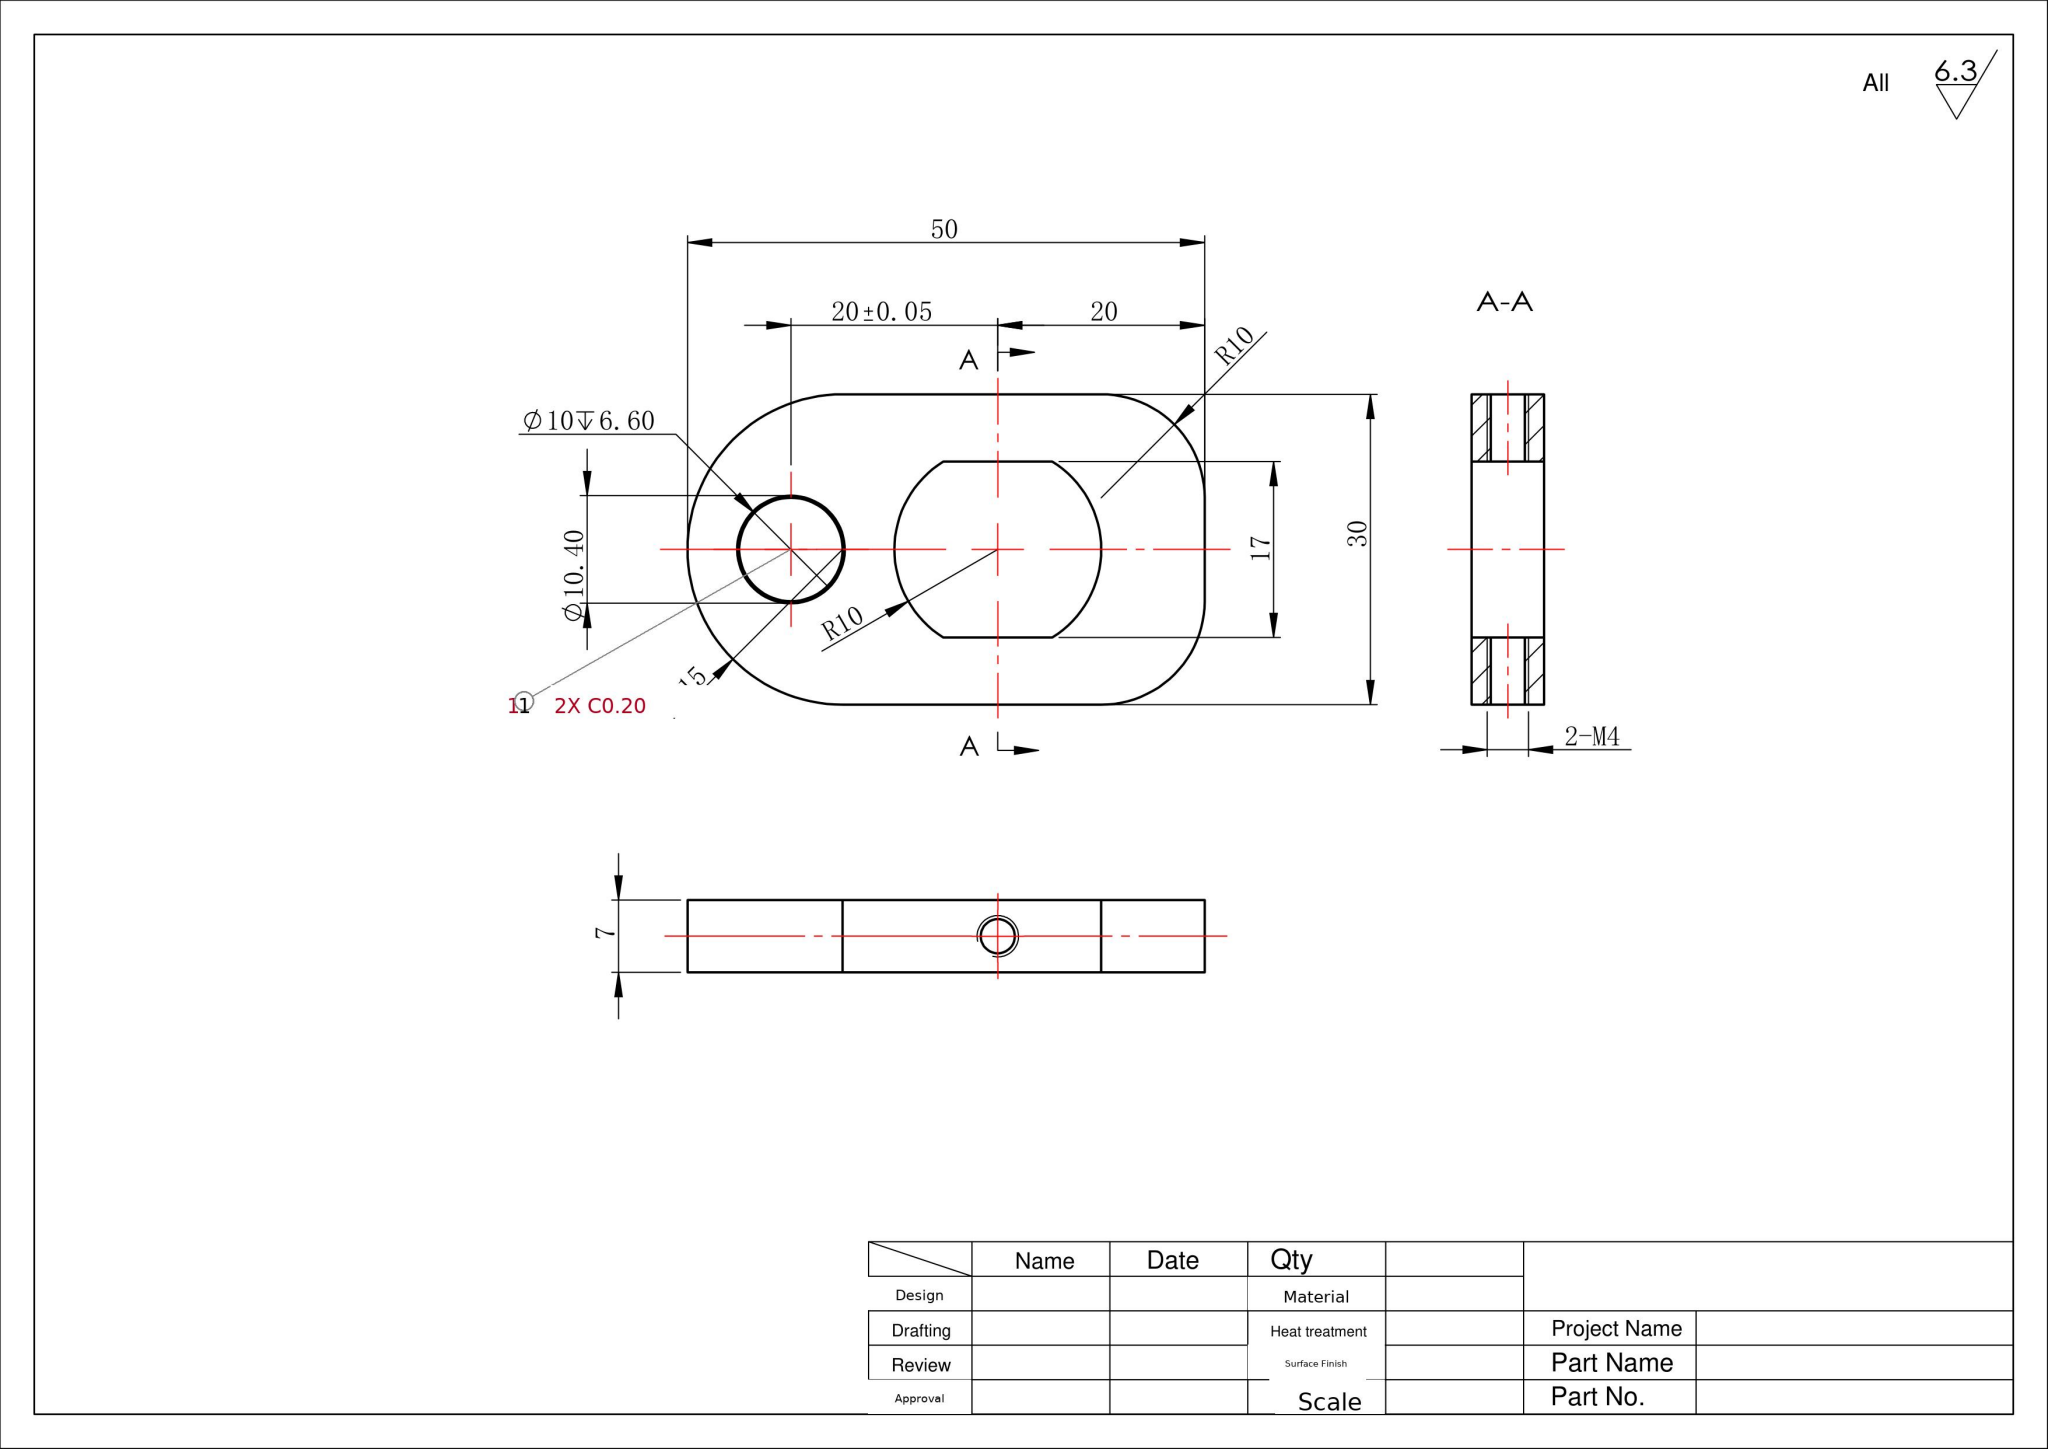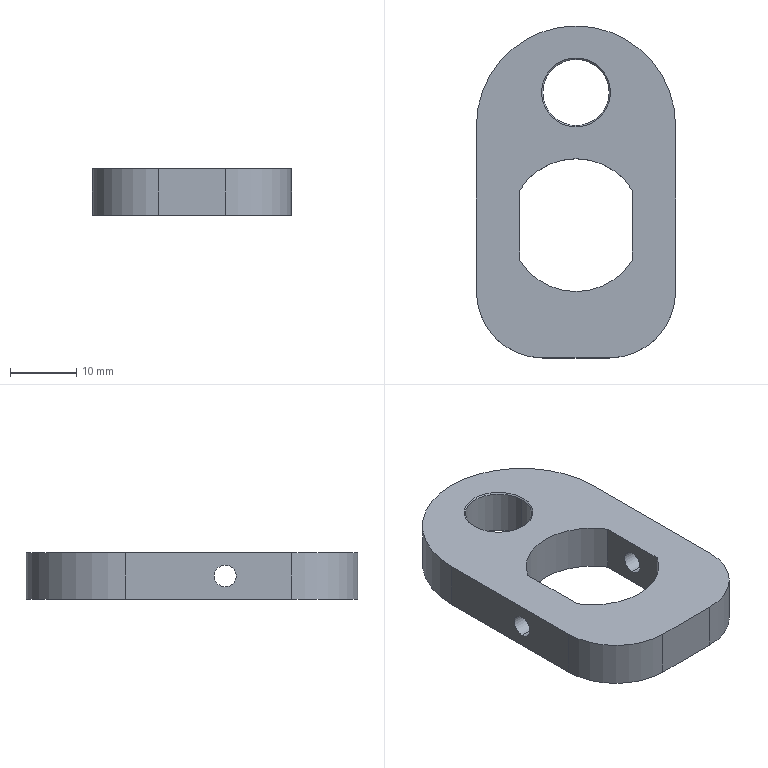Part | SolidWorks | mm | 1 solid | 23 faces | box 30 x 50 x 7 mm | volume 6812 mm3 | cylinder 12 | plane 7 | cone 4 | commonest cylinder face diameters 3.3 x4 20 x4 10 x2 30 x2
STEP:
#1=CARTESIAN_POINT('',(5.,20.,0.2));
#2=VERTEX_POINT('',#1);
#3=CARTESIAN_POINT('',(-5.,20.,0.2));
#4=VERTEX_POINT('',#3);
#5=CARTESIAN_POINT('',(-0.,20.,0.2));
#6=DIRECTION('',(0.,0.,-1.));
#7=DIRECTION('',(-1.,0.,0.));
#8=AXIS2_PLACEMENT_3D('',#5,#6,#7);
#9=CIRCLE('',#8,5.);
#10=EDGE_CURVE('',#2,#4,#9,.T.);
#11=ORIENTED_EDGE('',*,*,#10,.F.);
#12=CARTESIAN_POINT('',(5.2,20.,0.));
#13=VERTEX_POINT('',#12);
#14=CARTESIAN_POINT('',(5.,20.,0.2));
#15=DIRECTION('',(0.7071,0.,-0.7071));
#16=VECTOR('',#15,1000.);
#17=LINE('',#14,#16);
#18=EDGE_CURVE('',#2,#13,#17,.T.);
#19=ORIENTED_EDGE('',*,*,#18,.T.);
#20=CARTESIAN_POINT('',(-5.2,20.,0.));
#21=VERTEX_POINT('',#20);
#22=CARTESIAN_POINT('',(-0.,20.,0.));
#23=DIRECTION('',(0.,0.,1.));
#24=DIRECTION('',(-1.,0.,0.));
#25=AXIS2_PLACEMENT_3D('',#22,#23,#24);
#26=CIRCLE('',#25,5.2);
#27=EDGE_CURVE('',#21,#13,#26,.T.);
#28=ORIENTED_EDGE('',*,*,#27,.F.);
#29=CARTESIAN_POINT('',(-5.,20.,0.2));
#30=DIRECTION('',(-0.7071,0.,-0.7071));
#31=VECTOR('',#30,1000.);
#32=LINE('',#29,#31);
#33=EDGE_CURVE('',#4,#21,#32,.T.);
#34=ORIENTED_EDGE('',*,*,#33,.F.);
#35=EDGE_LOOP('',(#11,#19,#28,#34));
#36=FACE_OUTER_BOUND('',#35,.T.);
#37=CARTESIAN_POINT('',(-0.,20.,0.2));
#38=DIRECTION('',(0.,0.,-1.));
#39=DIRECTION('',(-1.,0.,0.));
#40=AXIS2_PLACEMENT_3D('',#37,#38,#39);
#41=CONICAL_SURFACE('',#40,5.,0.7854);
#42=ADVANCED_FACE('',(#36),#41,.F.);
#43=CARTESIAN_POINT('',(-5.,20.,6.8));
#44=VERTEX_POINT('',#43);
#45=CARTESIAN_POINT('',(5.,20.,6.8));
#46=VERTEX_POINT('',#45);
#47=CARTESIAN_POINT('',(-0.,20.,6.8));
#48=DIRECTION('',(0.,0.,1.));
#49=DIRECTION('',(-1.,0.,0.));
#50=AXIS2_PLACEMENT_3D('',#47,#48,#49);
#51=CIRCLE('',#50,5.);
#52=EDGE_CURVE('',#44,#46,#51,.T.);
#53=ORIENTED_EDGE('',*,*,#52,.F.);
#54=CARTESIAN_POINT('',(-5.2,20.,7.));
#55=VERTEX_POINT('',#54);
#56=CARTESIAN_POINT('',(-5.2,20.,7.));
#57=DIRECTION('',(-0.7071,0.,0.7071));
#58=VECTOR('',#57,1000.);
#59=LINE('',#56,#58);
#60=EDGE_CURVE('',#44,#55,#59,.T.);
#61=ORIENTED_EDGE('',*,*,#60,.T.);
#62=CARTESIAN_POINT('',(5.2,20.,7.));
#63=VERTEX_POINT('',#62);
#64=CARTESIAN_POINT('',(-0.,20.,7.));
#65=DIRECTION('',(0.,0.,-1.));
#66=DIRECTION('',(-1.,0.,0.));
#67=AXIS2_PLACEMENT_3D('',#64,#65,#66);
#68=CIRCLE('',#67,5.2);
#69=EDGE_CURVE('',#63,#55,#68,.T.);
#70=ORIENTED_EDGE('',*,*,#69,.F.);
#71=CARTESIAN_POINT('',(5.2,20.,7.));
#72=DIRECTION('',(0.7071,0.,0.7071));
#73=VECTOR('',#72,1000.);
#74=LINE('',#71,#73);
#75=EDGE_CURVE('',#46,#63,#74,.T.);
#76=ORIENTED_EDGE('',*,*,#75,.F.);
#77=EDGE_LOOP('',(#53,#61,#70,#76));
#78=FACE_OUTER_BOUND('',#77,.T.);
#79=CARTESIAN_POINT('',(-0.,20.,7.));
#80=DIRECTION('',(0.,0.,1.));
#81=DIRECTION('',(1.,0.,0.));
#82=AXIS2_PLACEMENT_3D('',#79,#80,#81);
#83=CONICAL_SURFACE('',#82,5.2,0.7854);
#84=ADVANCED_FACE('',(#78),#83,.F.);
#85=CARTESIAN_POINT('',(15.,0.,1.85));
#86=VERTEX_POINT('',#85);
#87=CARTESIAN_POINT('',(15.,0.,5.15));
#88=VERTEX_POINT('',#87);
#89=CARTESIAN_POINT('',(15.,0.,3.5));
#90=DIRECTION('',(-1.,0.,0.));
#91=DIRECTION('',(0.,0.,1.));
#92=AXIS2_PLACEMENT_3D('',#89,#90,#91);
#93=CIRCLE('',#92,1.65);
#94=EDGE_CURVE('',#86,#88,#93,.T.);
#95=ORIENTED_EDGE('',*,*,#94,.F.);
#96=CARTESIAN_POINT('',(8.5,0.,1.85));
#97=VERTEX_POINT('',#96);
#98=CARTESIAN_POINT('',(-15.,0.,1.85));
#99=DIRECTION('',(-1.,0.,0.));
#100=VECTOR('',#99,1000.);
#101=LINE('',#98,#100);
#102=EDGE_CURVE('',#86,#97,#101,.T.);
#103=ORIENTED_EDGE('',*,*,#102,.T.);
#104=CARTESIAN_POINT('',(8.5,0.,5.15));
#105=VERTEX_POINT('',#104);
#106=CARTESIAN_POINT('',(8.5,0.,3.5));
#107=DIRECTION('',(-1.,0.,0.));
#108=DIRECTION('',(0.,-1.,0.));
#109=AXIS2_PLACEMENT_3D('',#106,#107,#108);
#110=CIRCLE('',#109,1.65);
#111=EDGE_CURVE('',#97,#105,#110,.T.);
#112=ORIENTED_EDGE('',*,*,#111,.T.);
#113=CARTESIAN_POINT('',(-15.,0.,5.15));
#114=DIRECTION('',(-1.,0.,0.));
#115=VECTOR('',#114,1000.);
#116=LINE('',#113,#115);
#117=EDGE_CURVE('',#88,#105,#116,.T.);
#118=ORIENTED_EDGE('',*,*,#117,.F.);
#119=EDGE_LOOP('',(#95,#103,#112,#118));
#120=FACE_OUTER_BOUND('',#119,.T.);
#121=CARTESIAN_POINT('',(-15.,0.,3.5));
#122=DIRECTION('',(-1.,0.,0.));
#123=DIRECTION('',(0.,0.,1.));
#124=AXIS2_PLACEMENT_3D('',#121,#122,#123);
#125=CYLINDRICAL_SURFACE('',#124,1.65);
#126=ADVANCED_FACE('',(#120),#125,.F.);
#127=CARTESIAN_POINT('',(-8.5,0.,5.15));
#128=VERTEX_POINT('',#127);
#129=CARTESIAN_POINT('',(-8.5,0.,1.85));
#130=VERTEX_POINT('',#129);
#131=CARTESIAN_POINT('',(-8.5,0.,3.5));
#132=DIRECTION('',(1.,0.,0.));
#133=DIRECTION('',(0.,1.,0.));
#134=AXIS2_PLACEMENT_3D('',#131,#132,#133);
#135=CIRCLE('',#134,1.65);
#136=EDGE_CURVE('',#128,#130,#135,.T.);
#137=ORIENTED_EDGE('',*,*,#136,.T.);
#138=CARTESIAN_POINT('',(-15.,0.,1.85));
#139=VERTEX_POINT('',#138);
#140=CARTESIAN_POINT('',(-15.,0.,1.85));
#141=DIRECTION('',(-1.,0.,0.));
#142=VECTOR('',#141,1000.);
#143=LINE('',#140,#142);
#144=EDGE_CURVE('',#130,#139,#143,.T.);
#145=ORIENTED_EDGE('',*,*,#144,.T.);
#146=CARTESIAN_POINT('',(-15.,0.,5.15));
#147=VERTEX_POINT('',#146);
#148=CARTESIAN_POINT('',(-15.,0.,3.5));
#149=DIRECTION('',(-1.,0.,0.));
#150=DIRECTION('',(0.,0.,1.));
#151=AXIS2_PLACEMENT_3D('',#148,#149,#150);
#152=CIRCLE('',#151,1.65);
#153=EDGE_CURVE('',#139,#147,#152,.T.);
#154=ORIENTED_EDGE('',*,*,#153,.T.);
#155=CARTESIAN_POINT('',(-15.,0.,5.15));
#156=DIRECTION('',(-1.,0.,0.));
#157=VECTOR('',#156,1000.);
#158=LINE('',#155,#157);
#159=EDGE_CURVE('',#128,#147,#158,.T.);
#160=ORIENTED_EDGE('',*,*,#159,.F.);
#161=EDGE_LOOP('',(#137,#145,#154,#160));
#162=FACE_OUTER_BOUND('',#161,.T.);
#163=CARTESIAN_POINT('',(-15.,0.,3.5));
#164=DIRECTION('',(-1.,0.,0.));
#165=DIRECTION('',(0.,0.,1.));
#166=AXIS2_PLACEMENT_3D('',#163,#164,#165);
#167=CYLINDRICAL_SURFACE('',#166,1.65);
#168=ADVANCED_FACE('',(#162),#167,.F.);
#169=ORIENTED_EDGE('',*,*,#52,.T.);
#170=CARTESIAN_POINT('',(5.,20.,7.));
#171=DIRECTION('',(0.,0.,-1.));
#172=VECTOR('',#171,1000.);
#173=LINE('',#170,#172);
#174=EDGE_CURVE('',#46,#2,#173,.T.);
#175=ORIENTED_EDGE('',*,*,#174,.T.);
#176=ORIENTED_EDGE('',*,*,#10,.T.);
#177=CARTESIAN_POINT('',(-5.,20.,7.));
#178=DIRECTION('',(0.,0.,-1.));
#179=VECTOR('',#178,1000.);
#180=LINE('',#177,#179);
#181=EDGE_CURVE('',#44,#4,#180,.T.);
#182=ORIENTED_EDGE('',*,*,#181,.F.);
#183=EDGE_LOOP('',(#169,#175,#176,#182));
#184=FACE_OUTER_BOUND('',#183,.T.);
#185=CARTESIAN_POINT('',(-0.,20.,7.));
#186=DIRECTION('',(0.,0.,-1.));
#187=DIRECTION('',(-1.,0.,0.));
#188=AXIS2_PLACEMENT_3D('',#185,#186,#187);
#189=CYLINDRICAL_SURFACE('',#188,5.);
#190=ADVANCED_FACE('',(#184),#189,.F.);
#191=ORIENTED_EDGE('',*,*,#69,.T.);
#192=CARTESIAN_POINT('',(-0.,20.,7.));
#193=DIRECTION('',(0.,0.,-1.));
#194=DIRECTION('',(-1.,0.,0.));
#195=AXIS2_PLACEMENT_3D('',#192,#193,#194);
#196=CIRCLE('',#195,5.2);
#197=EDGE_CURVE('',#55,#63,#196,.T.);
#198=ORIENTED_EDGE('',*,*,#197,.T.);
#199=EDGE_LOOP('',(#191,#198));
#200=FACE_BOUND('',#199,.T.);
#201=CARTESIAN_POINT('',(-15.,15.,7.));
#202=VERTEX_POINT('',#201);
#203=CARTESIAN_POINT('',(-15.,-10.,7.));
#204=VERTEX_POINT('',#203);
#205=CARTESIAN_POINT('',(-15.,-30.,7.));
#206=DIRECTION('',(0.,-1.,0.));
#207=VECTOR('',#206,1000.);
#208=LINE('',#205,#207);
#209=EDGE_CURVE('',#202,#204,#208,.T.);
#210=ORIENTED_EDGE('',*,*,#209,.T.);
#211=CARTESIAN_POINT('',(-5.,-20.,7.));
#212=VERTEX_POINT('',#211);
#213=CARTESIAN_POINT('',(-5.,-10.,7.));
#214=DIRECTION('',(0.,0.,1.));
#215=DIRECTION('',(-1.,0.,0.));
#216=AXIS2_PLACEMENT_3D('',#213,#214,#215);
#217=CIRCLE('',#216,10.);
#218=EDGE_CURVE('',#204,#212,#217,.T.);
#219=ORIENTED_EDGE('',*,*,#218,.T.);
#220=CARTESIAN_POINT('',(5.,-20.,7.));
#221=VERTEX_POINT('',#220);
#222=CARTESIAN_POINT('',(29.445,-20.,7.));
#223=DIRECTION('',(1.,0.,0.));
#224=VECTOR('',#223,1000.);
#225=LINE('',#222,#224);
#226=EDGE_CURVE('',#212,#221,#225,.T.);
#227=ORIENTED_EDGE('',*,*,#226,.T.);
#228=CARTESIAN_POINT('',(15.,-10.,7.));
#229=VERTEX_POINT('',#228);
#230=CARTESIAN_POINT('',(5.,-10.,7.));
#231=DIRECTION('',(0.,0.,1.));
#232=DIRECTION('',(-1.,0.,0.));
#233=AXIS2_PLACEMENT_3D('',#230,#231,#232);
#234=CIRCLE('',#233,10.);
#235=EDGE_CURVE('',#221,#229,#234,.T.);
#236=ORIENTED_EDGE('',*,*,#235,.T.);
#237=CARTESIAN_POINT('',(15.,15.,7.));
#238=VERTEX_POINT('',#237);
#239=CARTESIAN_POINT('',(15.,-30.,7.));
#240=DIRECTION('',(0.,1.,0.));
#241=VECTOR('',#240,1000.);
#242=LINE('',#239,#241);
#243=EDGE_CURVE('',#229,#238,#242,.T.);
#244=ORIENTED_EDGE('',*,*,#243,.T.);
#245=CARTESIAN_POINT('',(0.,30.,7.));
#246=VERTEX_POINT('',#245);
#247=CARTESIAN_POINT('',(0.,15.,7.));
#248=DIRECTION('',(0.,0.,1.));
#249=DIRECTION('',(-1.,0.,0.));
#250=AXIS2_PLACEMENT_3D('',#247,#248,#249);
#251=CIRCLE('',#250,15.);
#252=EDGE_CURVE('',#238,#246,#251,.T.);
#253=ORIENTED_EDGE('',*,*,#252,.T.);
#254=CARTESIAN_POINT('',(0.,15.,7.));
#255=DIRECTION('',(0.,0.,1.));
#256=DIRECTION('',(-1.,0.,0.));
#257=AXIS2_PLACEMENT_3D('',#254,#255,#256);
#258=CIRCLE('',#257,15.);
#259=EDGE_CURVE('',#246,#202,#258,.T.);
#260=ORIENTED_EDGE('',*,*,#259,.T.);
#261=EDGE_LOOP('',(#210,#219,#227,#236,#244,#253,#260));
#262=FACE_OUTER_BOUND('',#261,.T.);
#263=CARTESIAN_POINT('',(-8.5,-5.268,7.));
#264=VERTEX_POINT('',#263);
#265=CARTESIAN_POINT('',(8.5,-5.268,7.));
#266=VERTEX_POINT('',#265);
#267=CARTESIAN_POINT('',(0.,0.,7.));
#268=DIRECTION('',(0.,0.,1.));
#269=DIRECTION('',(1.,0.,0.));
#270=AXIS2_PLACEMENT_3D('',#267,#268,#269);
#271=CIRCLE('',#270,10.);
#272=EDGE_CURVE('',#264,#266,#271,.T.);
#273=ORIENTED_EDGE('',*,*,#272,.F.);
#274=CARTESIAN_POINT('',(-8.5,5.268,7.));
#275=VERTEX_POINT('',#274);
#276=CARTESIAN_POINT('',(-8.5,-5.268,7.));
#277=DIRECTION('',(0.,-1.,0.));
#278=VECTOR('',#277,1000.);
#279=LINE('',#276,#278);
#280=EDGE_CURVE('',#275,#264,#279,.T.);
#281=ORIENTED_EDGE('',*,*,#280,.F.);
#282=CARTESIAN_POINT('',(8.5,5.268,7.));
#283=VERTEX_POINT('',#282);
#284=CARTESIAN_POINT('',(0.,0.,7.));
#285=DIRECTION('',(0.,0.,1.));
#286=DIRECTION('',(1.,0.,0.));
#287=AXIS2_PLACEMENT_3D('',#284,#285,#286);
#288=CIRCLE('',#287,10.);
#289=EDGE_CURVE('',#283,#275,#288,.T.);
#290=ORIENTED_EDGE('',*,*,#289,.F.);
#291=CARTESIAN_POINT('',(8.5,-5.268,7.));
#292=DIRECTION('',(0.,1.,0.));
#293=VECTOR('',#292,1000.);
#294=LINE('',#291,#293);
#295=EDGE_CURVE('',#266,#283,#294,.T.);
#296=ORIENTED_EDGE('',*,*,#295,.F.);
#297=EDGE_LOOP('',(#273,#281,#290,#296));
#298=FACE_BOUND('',#297,.T.);
#299=CARTESIAN_POINT('',(-15.,30.,7.));
#300=DIRECTION('',(0.,0.,-1.));
#301=DIRECTION('',(-1.,0.,0.));
#302=AXIS2_PLACEMENT_3D('',#299,#300,#301);
#303=PLANE('',#302);
#304=ADVANCED_FACE('',(#200,#262,#298),#303,.F.);
#305=ORIENTED_EDGE('',*,*,#27,.T.);
#306=CARTESIAN_POINT('',(-0.,20.,0.));
#307=DIRECTION('',(0.,0.,1.));
#308=DIRECTION('',(-1.,0.,0.));
#309=AXIS2_PLACEMENT_3D('',#306,#307,#308);
#310=CIRCLE('',#309,5.2);
#311=EDGE_CURVE('',#13,#21,#310,.T.);
#312=ORIENTED_EDGE('',*,*,#311,.T.);
#313=EDGE_LOOP('',(#305,#312));
#314=FACE_BOUND('',#313,.T.);
#315=CARTESIAN_POINT('',(-5.,-20.,0.));
#316=VERTEX_POINT('',#315);
#317=CARTESIAN_POINT('',(5.,-20.,0.));
#318=VERTEX_POINT('',#317);
#319=CARTESIAN_POINT('',(29.445,-20.,0.));
#320=DIRECTION('',(1.,0.,0.));
#321=VECTOR('',#320,1000.);
#322=LINE('',#319,#321);
#323=EDGE_CURVE('',#316,#318,#322,.T.);
#324=ORIENTED_EDGE('',*,*,#323,.F.);
#325=CARTESIAN_POINT('',(-15.,-10.,0.));
#326=VERTEX_POINT('',#325);
#327=CARTESIAN_POINT('',(-5.,-10.,0.));
#328=DIRECTION('',(0.,0.,-1.));
#329=DIRECTION('',(-1.,0.,0.));
#330=AXIS2_PLACEMENT_3D('',#327,#328,#329);
#331=CIRCLE('',#330,10.);
#332=EDGE_CURVE('',#316,#326,#331,.T.);
#333=ORIENTED_EDGE('',*,*,#332,.T.);
#334=CARTESIAN_POINT('',(-15.,15.,0.));
#335=VERTEX_POINT('',#334);
#336=CARTESIAN_POINT('',(-15.,-30.,0.));
#337=DIRECTION('',(0.,-1.,0.));
#338=VECTOR('',#337,1000.);
#339=LINE('',#336,#338);
#340=EDGE_CURVE('',#335,#326,#339,.T.);
#341=ORIENTED_EDGE('',*,*,#340,.F.);
#342=CARTESIAN_POINT('',(0.,30.,0.));
#343=VERTEX_POINT('',#342);
#344=CARTESIAN_POINT('',(0.,15.,0.));
#345=DIRECTION('',(0.,0.,-1.));
#346=DIRECTION('',(-1.,0.,0.));
#347=AXIS2_PLACEMENT_3D('',#344,#345,#346);
#348=CIRCLE('',#347,15.);
#349=EDGE_CURVE('',#335,#343,#348,.T.);
#350=ORIENTED_EDGE('',*,*,#349,.T.);
#351=CARTESIAN_POINT('',(15.,15.,0.));
#352=VERTEX_POINT('',#351);
#353=CARTESIAN_POINT('',(0.,15.,0.));
#354=DIRECTION('',(0.,0.,-1.));
#355=DIRECTION('',(-1.,0.,0.));
#356=AXIS2_PLACEMENT_3D('',#353,#354,#355);
#357=CIRCLE('',#356,15.);
#358=EDGE_CURVE('',#343,#352,#357,.T.);
#359=ORIENTED_EDGE('',*,*,#358,.T.);
#360=CARTESIAN_POINT('',(15.,-10.,0.));
#361=VERTEX_POINT('',#360);
#362=CARTESIAN_POINT('',(15.,-30.,0.));
#363=DIRECTION('',(0.,1.,0.));
#364=VECTOR('',#363,1000.);
#365=LINE('',#362,#364);
#366=EDGE_CURVE('',#361,#352,#365,.T.);
#367=ORIENTED_EDGE('',*,*,#366,.F.);
#368=CARTESIAN_POINT('',(5.,-10.,0.));
#369=DIRECTION('',(0.,0.,-1.));
#370=DIRECTION('',(-1.,0.,0.));
#371=AXIS2_PLACEMENT_3D('',#368,#369,#370);
#372=CIRCLE('',#371,10.);
#373=EDGE_CURVE('',#361,#318,#372,.T.);
#374=ORIENTED_EDGE('',*,*,#373,.T.);
#375=EDGE_LOOP('',(#324,#333,#341,#350,#359,#367,#374));
#376=FACE_OUTER_BOUND('',#375,.T.);
#377=CARTESIAN_POINT('',(-8.5,5.268,0.));
#378=VERTEX_POINT('',#377);
#379=CARTESIAN_POINT('',(-8.5,-5.268,0.));
#380=VERTEX_POINT('',#379);
#381=CARTESIAN_POINT('',(-8.5,-5.268,0.));
#382=DIRECTION('',(0.,-1.,0.));
#383=VECTOR('',#382,1000.);
#384=LINE('',#381,#383);
#385=EDGE_CURVE('',#378,#380,#384,.T.);
#386=ORIENTED_EDGE('',*,*,#385,.T.);
#387=CARTESIAN_POINT('',(8.5,-5.268,0.));
#388=VERTEX_POINT('',#387);
#389=CARTESIAN_POINT('',(0.,0.,0.));
#390=DIRECTION('',(0.,0.,1.));
#391=DIRECTION('',(1.,0.,0.));
#392=AXIS2_PLACEMENT_3D('',#389,#390,#391);
#393=CIRCLE('',#392,10.);
#394=EDGE_CURVE('',#380,#388,#393,.T.);
#395=ORIENTED_EDGE('',*,*,#394,.T.);
#396=CARTESIAN_POINT('',(8.5,5.268,0.));
#397=VERTEX_POINT('',#396);
#398=CARTESIAN_POINT('',(8.5,-5.268,0.));
#399=DIRECTION('',(0.,1.,0.));
#400=VECTOR('',#399,1000.);
#401=LINE('',#398,#400);
#402=EDGE_CURVE('',#388,#397,#401,.T.);
#403=ORIENTED_EDGE('',*,*,#402,.T.);
#404=CARTESIAN_POINT('',(0.,0.,0.));
#405=DIRECTION('',(0.,0.,1.));
#406=DIRECTION('',(1.,0.,0.));
#407=AXIS2_PLACEMENT_3D('',#404,#405,#406);
#408=CIRCLE('',#407,10.);
#409=EDGE_CURVE('',#397,#378,#408,.T.);
#410=ORIENTED_EDGE('',*,*,#409,.T.);
#411=EDGE_LOOP('',(#386,#395,#403,#410));
#412=FACE_BOUND('',#411,.T.);
#413=CARTESIAN_POINT('',(-15.,30.,0.));
#414=DIRECTION('',(0.,0.,-1.));
#415=DIRECTION('',(-1.,0.,0.));
#416=AXIS2_PLACEMENT_3D('',#413,#414,#415);
#417=PLANE('',#416);
#418=ADVANCED_FACE('',(#314,#376,#412),#417,.T.);
#419=CARTESIAN_POINT('',(-15.,0.,3.5));
#420=DIRECTION('',(-1.,0.,0.));
#421=DIRECTION('',(0.,0.,1.));
#422=AXIS2_PLACEMENT_3D('',#419,#420,#421);
#423=CIRCLE('',#422,1.65);
#424=EDGE_CURVE('',#147,#139,#423,.T.);
#425=ORIENTED_EDGE('',*,*,#424,.F.);
#426=ORIENTED_EDGE('',*,*,#153,.F.);
#427=EDGE_LOOP('',(#425,#426));
#428=FACE_BOUND('',#427,.T.);
#429=ORIENTED_EDGE('',*,*,#340,.T.);
#430=CARTESIAN_POINT('',(-15.,-10.,7.));
#431=DIRECTION('',(0.,0.,1.));
#432=VECTOR('',#431,1000.);
#433=LINE('',#430,#432);
#434=EDGE_CURVE('',#326,#204,#433,.T.);
#435=ORIENTED_EDGE('',*,*,#434,.T.);
#436=ORIENTED_EDGE('',*,*,#209,.F.);
#437=CARTESIAN_POINT('',(-15.,15.,7.));
#438=DIRECTION('',(0.,0.,-1.));
#439=VECTOR('',#438,1000.);
#440=LINE('',#437,#439);
#441=EDGE_CURVE('',#202,#335,#440,.T.);
#442=ORIENTED_EDGE('',*,*,#441,.T.);
#443=EDGE_LOOP('',(#429,#435,#436,#442));
#444=FACE_OUTER_BOUND('',#443,.T.);
#445=CARTESIAN_POINT('',(-15.,-30.,7.));
#446=DIRECTION('',(1.,0.,0.));
#447=DIRECTION('',(0.,0.,-1.));
#448=AXIS2_PLACEMENT_3D('',#445,#446,#447);
#449=PLANE('',#448);
#450=ADVANCED_FACE('',(#428,#444),#449,.F.);
#451=CARTESIAN_POINT('',(15.,0.,3.5));
#452=DIRECTION('',(-1.,0.,0.));
#453=DIRECTION('',(0.,0.,1.));
#454=AXIS2_PLACEMENT_3D('',#451,#452,#453);
#455=CIRCLE('',#454,1.65);
#456=EDGE_CURVE('',#88,#86,#455,.T.);
#457=ORIENTED_EDGE('',*,*,#456,.T.);
#458=ORIENTED_EDGE('',*,*,#94,.T.);
#459=EDGE_LOOP('',(#457,#458));
#460=FACE_BOUND('',#459,.T.);
#461=ORIENTED_EDGE('',*,*,#243,.F.);
#462=CARTESIAN_POINT('',(15.,-10.,7.));
#463=DIRECTION('',(0.,0.,-1.));
#464=VECTOR('',#463,1000.);
#465=LINE('',#462,#464);
#466=EDGE_CURVE('',#229,#361,#465,.T.);
#467=ORIENTED_EDGE('',*,*,#466,.T.);
#468=ORIENTED_EDGE('',*,*,#366,.T.);
#469=CARTESIAN_POINT('',(15.,15.,7.));
#470=DIRECTION('',(0.,0.,1.));
#471=VECTOR('',#470,1000.);
#472=LINE('',#469,#471);
#473=EDGE_CURVE('',#352,#238,#472,.T.);
#474=ORIENTED_EDGE('',*,*,#473,.T.);
#475=EDGE_LOOP('',(#461,#467,#468,#474));
#476=FACE_OUTER_BOUND('',#475,.T.);
#477=CARTESIAN_POINT('',(15.,-30.,7.));
#478=DIRECTION('',(-1.,0.,0.));
#479=DIRECTION('',(0.,0.,1.));
#480=AXIS2_PLACEMENT_3D('',#477,#478,#479);
#481=PLANE('',#480);
#482=ADVANCED_FACE('',(#460,#476),#481,.F.);
#483=ORIENTED_EDGE('',*,*,#394,.F.);
#484=CARTESIAN_POINT('',(-8.5,-5.268,7.));
#485=DIRECTION('',(0.,0.,-1.));
#486=VECTOR('',#485,1000.);
#487=LINE('',#484,#486);
#488=EDGE_CURVE('',#264,#380,#487,.T.);
#489=ORIENTED_EDGE('',*,*,#488,.F.);
#490=ORIENTED_EDGE('',*,*,#272,.T.);
#491=CARTESIAN_POINT('',(8.5,-5.268,7.));
#492=DIRECTION('',(0.,0.,-1.));
#493=VECTOR('',#492,1000.);
#494=LINE('',#491,#493);
#495=EDGE_CURVE('',#266,#388,#494,.T.);
#496=ORIENTED_EDGE('',*,*,#495,.T.);
#497=EDGE_LOOP('',(#483,#489,#490,#496));
#498=FACE_OUTER_BOUND('',#497,.T.);
#499=CARTESIAN_POINT('',(0.,0.,7.));
#500=DIRECTION('',(0.,0.,-1.));
#501=DIRECTION('',(-1.,0.,0.));
#502=AXIS2_PLACEMENT_3D('',#499,#500,#501);
#503=CYLINDRICAL_SURFACE('',#502,10.);
#504=ADVANCED_FACE('',(#498),#503,.F.);
#505=CARTESIAN_POINT('',(8.5,0.,3.5));
#506=DIRECTION('',(-1.,0.,0.));
#507=DIRECTION('',(0.,-1.,0.));
#508=AXIS2_PLACEMENT_3D('',#505,#506,#507);
#509=CIRCLE('',#508,1.65);
#510=EDGE_CURVE('',#105,#97,#509,.T.);
#511=ORIENTED_EDGE('',*,*,#510,.F.);
#512=ORIENTED_EDGE('',*,*,#111,.F.);
#513=EDGE_LOOP('',(#511,#512));
#514=FACE_BOUND('',#513,.T.);
#515=ORIENTED_EDGE('',*,*,#402,.F.);
#516=ORIENTED_EDGE('',*,*,#495,.F.);
#517=ORIENTED_EDGE('',*,*,#295,.T.);
#518=CARTESIAN_POINT('',(8.5,5.268,7.));
#519=DIRECTION('',(0.,0.,-1.));
#520=VECTOR('',#519,1000.);
#521=LINE('',#518,#520);
#522=EDGE_CURVE('',#283,#397,#521,.T.);
#523=ORIENTED_EDGE('',*,*,#522,.T.);
#524=EDGE_LOOP('',(#515,#516,#517,#523));
#525=FACE_OUTER_BOUND('',#524,.T.);
#526=CARTESIAN_POINT('',(8.5,-5.268,7.));
#527=DIRECTION('',(-1.,0.,0.));
#528=DIRECTION('',(-0.,-1.,0.));
#529=AXIS2_PLACEMENT_3D('',#526,#527,#528);
#530=PLANE('',#529);
#531=ADVANCED_FACE('',(#514,#525),#530,.T.);
#532=ORIENTED_EDGE('',*,*,#409,.F.);
#533=ORIENTED_EDGE('',*,*,#522,.F.);
#534=ORIENTED_EDGE('',*,*,#289,.T.);
#535=CARTESIAN_POINT('',(-8.5,5.268,7.));
#536=DIRECTION('',(0.,0.,-1.));
#537=VECTOR('',#536,1000.);
#538=LINE('',#535,#537);
#539=EDGE_CURVE('',#275,#378,#538,.T.);
#540=ORIENTED_EDGE('',*,*,#539,.T.);
#541=EDGE_LOOP('',(#532,#533,#534,#540));
#542=FACE_OUTER_BOUND('',#541,.T.);
#543=CARTESIAN_POINT('',(0.,0.,7.));
#544=DIRECTION('',(0.,0.,-1.));
#545=DIRECTION('',(-1.,0.,0.));
#546=AXIS2_PLACEMENT_3D('',#543,#544,#545);
#547=CYLINDRICAL_SURFACE('',#546,10.);
#548=ADVANCED_FACE('',(#542),#547,.F.);
#549=ORIENTED_EDGE('',*,*,#136,.F.);
#550=CARTESIAN_POINT('',(-8.5,0.,3.5));
#551=DIRECTION('',(1.,0.,0.));
#552=DIRECTION('',(0.,1.,0.));
#553=AXIS2_PLACEMENT_3D('',#550,#551,#552);
#554=CIRCLE('',#553,1.65);
#555=EDGE_CURVE('',#130,#128,#554,.T.);
#556=ORIENTED_EDGE('',*,*,#555,.F.);
#557=EDGE_LOOP('',(#549,#556));
#558=FACE_BOUND('',#557,.T.);
#559=ORIENTED_EDGE('',*,*,#385,.F.);
#560=ORIENTED_EDGE('',*,*,#539,.F.);
#561=ORIENTED_EDGE('',*,*,#280,.T.);
#562=ORIENTED_EDGE('',*,*,#488,.T.);
#563=EDGE_LOOP('',(#559,#560,#561,#562));
#564=FACE_OUTER_BOUND('',#563,.T.);
#565=CARTESIAN_POINT('',(-8.5,-5.268,7.));
#566=DIRECTION('',(1.,0.,0.));
#567=DIRECTION('',(-0.,1.,0.));
#568=AXIS2_PLACEMENT_3D('',#565,#566,#567);
#569=PLANE('',#568);
#570=ADVANCED_FACE('',(#558,#564),#569,.T.);
#571=ORIENTED_EDGE('',*,*,#174,.F.);
#572=CARTESIAN_POINT('',(-0.,20.,6.8));
#573=DIRECTION('',(0.,0.,1.));
#574=DIRECTION('',(-1.,0.,0.));
#575=AXIS2_PLACEMENT_3D('',#572,#573,#574);
#576=CIRCLE('',#575,5.);
#577=EDGE_CURVE('',#46,#44,#576,.T.);
#578=ORIENTED_EDGE('',*,*,#577,.T.);
#579=ORIENTED_EDGE('',*,*,#181,.T.);
#580=CARTESIAN_POINT('',(-0.,20.,0.2));
#581=DIRECTION('',(0.,0.,-1.));
#582=DIRECTION('',(-1.,0.,0.));
#583=AXIS2_PLACEMENT_3D('',#580,#581,#582);
#584=CIRCLE('',#583,5.);
#585=EDGE_CURVE('',#4,#2,#584,.T.);
#586=ORIENTED_EDGE('',*,*,#585,.T.);
#587=EDGE_LOOP('',(#571,#578,#579,#586));
#588=FACE_OUTER_BOUND('',#587,.T.);
#589=CARTESIAN_POINT('',(-0.,20.,7.));
#590=DIRECTION('',(0.,0.,-1.));
#591=DIRECTION('',(-1.,0.,0.));
#592=AXIS2_PLACEMENT_3D('',#589,#590,#591);
#593=CYLINDRICAL_SURFACE('',#592,5.);
#594=ADVANCED_FACE('',(#588),#593,.F.);
#595=ORIENTED_EDGE('',*,*,#226,.F.);
#596=CARTESIAN_POINT('',(-5.,-20.,7.));
#597=DIRECTION('',(0.,0.,-1.));
#598=VECTOR('',#597,1000.);
#599=LINE('',#596,#598);
#600=EDGE_CURVE('',#212,#316,#599,.T.);
#601=ORIENTED_EDGE('',*,*,#600,.T.);
#602=ORIENTED_EDGE('',*,*,#323,.T.);
#603=CARTESIAN_POINT('',(5.,-20.,7.));
#604=DIRECTION('',(0.,0.,1.));
#605=VECTOR('',#604,1000.);
#606=LINE('',#603,#605);
#607=EDGE_CURVE('',#318,#221,#606,.T.);
#608=ORIENTED_EDGE('',*,*,#607,.T.);
#609=EDGE_LOOP('',(#595,#601,#602,#608));
#610=FACE_OUTER_BOUND('',#609,.T.);
#611=CARTESIAN_POINT('',(29.445,-20.,7.));
#612=DIRECTION('',(0.,1.,0.));
#613=DIRECTION('',(0.,0.,1.));
#614=AXIS2_PLACEMENT_3D('',#611,#612,#613);
#615=PLANE('',#614);
#616=ADVANCED_FACE('',(#610),#615,.F.);
#617=ORIENTED_EDGE('',*,*,#252,.F.);
#618=ORIENTED_EDGE('',*,*,#473,.F.);
#619=ORIENTED_EDGE('',*,*,#358,.F.);
#620=CARTESIAN_POINT('',(0.,30.,7.));
#621=DIRECTION('',(0.,0.,-1.));
#622=VECTOR('',#621,1000.);
#623=LINE('',#620,#622);
#624=EDGE_CURVE('',#246,#343,#623,.T.);
#625=ORIENTED_EDGE('',*,*,#624,.F.);
#626=EDGE_LOOP('',(#617,#618,#619,#625));
#627=FACE_OUTER_BOUND('',#626,.T.);
#628=CARTESIAN_POINT('',(0.,15.,7.));
#629=DIRECTION('',(0.,0.,-1.));
#630=DIRECTION('',(-1.,0.,0.));
#631=AXIS2_PLACEMENT_3D('',#628,#629,#630);
#632=CYLINDRICAL_SURFACE('',#631,15.);
#633=ADVANCED_FACE('',(#627),#632,.T.);
#634=ORIENTED_EDGE('',*,*,#259,.F.);
#635=ORIENTED_EDGE('',*,*,#624,.T.);
#636=ORIENTED_EDGE('',*,*,#349,.F.);
#637=ORIENTED_EDGE('',*,*,#441,.F.);
#638=EDGE_LOOP('',(#634,#635,#636,#637));
#639=FACE_OUTER_BOUND('',#638,.T.);
#640=CARTESIAN_POINT('',(0.,15.,7.));
#641=DIRECTION('',(0.,0.,-1.));
#642=DIRECTION('',(-1.,0.,0.));
#643=AXIS2_PLACEMENT_3D('',#640,#641,#642);
#644=CYLINDRICAL_SURFACE('',#643,15.);
#645=ADVANCED_FACE('',(#639),#644,.T.);
#646=ORIENTED_EDGE('',*,*,#332,.F.);
#647=ORIENTED_EDGE('',*,*,#600,.F.);
#648=ORIENTED_EDGE('',*,*,#218,.F.);
#649=ORIENTED_EDGE('',*,*,#434,.F.);
#650=EDGE_LOOP('',(#646,#647,#648,#649));
#651=FACE_OUTER_BOUND('',#650,.T.);
#652=CARTESIAN_POINT('',(-5.,-10.,7.));
#653=DIRECTION('',(0.,0.,1.));
#654=DIRECTION('',(1.,0.,0.));
#655=AXIS2_PLACEMENT_3D('',#652,#653,#654);
#656=CYLINDRICAL_SURFACE('',#655,10.);
#657=ADVANCED_FACE('',(#651),#656,.T.);
#658=ORIENTED_EDGE('',*,*,#235,.F.);
#659=ORIENTED_EDGE('',*,*,#607,.F.);
#660=ORIENTED_EDGE('',*,*,#373,.F.);
#661=ORIENTED_EDGE('',*,*,#466,.F.);
#662=EDGE_LOOP('',(#658,#659,#660,#661));
#663=FACE_OUTER_BOUND('',#662,.T.);
#664=CARTESIAN_POINT('',(5.,-10.,7.));
#665=DIRECTION('',(0.,0.,-1.));
#666=DIRECTION('',(-1.,0.,0.));
#667=AXIS2_PLACEMENT_3D('',#664,#665,#666);
#668=CYLINDRICAL_SURFACE('',#667,10.);
#669=ADVANCED_FACE('',(#663),#668,.T.);
#670=ORIENTED_EDGE('',*,*,#144,.F.);
#671=ORIENTED_EDGE('',*,*,#555,.T.);
#672=ORIENTED_EDGE('',*,*,#159,.T.);
#673=ORIENTED_EDGE('',*,*,#424,.T.);
#674=EDGE_LOOP('',(#670,#671,#672,#673));
#675=FACE_OUTER_BOUND('',#674,.T.);
#676=CARTESIAN_POINT('',(-15.,0.,3.5));
#677=DIRECTION('',(-1.,0.,0.));
#678=DIRECTION('',(0.,0.,1.));
#679=AXIS2_PLACEMENT_3D('',#676,#677,#678);
#680=CYLINDRICAL_SURFACE('',#679,1.65);
#681=ADVANCED_FACE('',(#675),#680,.F.);
#682=ORIENTED_EDGE('',*,*,#102,.F.);
#683=ORIENTED_EDGE('',*,*,#456,.F.);
#684=ORIENTED_EDGE('',*,*,#117,.T.);
#685=ORIENTED_EDGE('',*,*,#510,.T.);
#686=EDGE_LOOP('',(#682,#683,#684,#685));
#687=FACE_OUTER_BOUND('',#686,.T.);
#688=CARTESIAN_POINT('',(-15.,0.,3.5));
#689=DIRECTION('',(-1.,0.,0.));
#690=DIRECTION('',(0.,0.,1.));
#691=AXIS2_PLACEMENT_3D('',#688,#689,#690);
#692=CYLINDRICAL_SURFACE('',#691,1.65);
#693=ADVANCED_FACE('',(#687),#692,.F.);
#694=ORIENTED_EDGE('',*,*,#60,.F.);
#695=ORIENTED_EDGE('',*,*,#577,.F.);
#696=ORIENTED_EDGE('',*,*,#75,.T.);
#697=ORIENTED_EDGE('',*,*,#197,.F.);
#698=EDGE_LOOP('',(#694,#695,#696,#697));
#699=FACE_OUTER_BOUND('',#698,.T.);
#700=CARTESIAN_POINT('',(-0.,20.,7.));
#701=DIRECTION('',(0.,0.,1.));
#702=DIRECTION('',(1.,0.,0.));
#703=AXIS2_PLACEMENT_3D('',#700,#701,#702);
#704=CONICAL_SURFACE('',#703,5.2,0.7854);
#705=ADVANCED_FACE('',(#699),#704,.F.);
#706=ORIENTED_EDGE('',*,*,#18,.F.);
#707=ORIENTED_EDGE('',*,*,#585,.F.);
#708=ORIENTED_EDGE('',*,*,#33,.T.);
#709=ORIENTED_EDGE('',*,*,#311,.F.);
#710=EDGE_LOOP('',(#706,#707,#708,#709));
#711=FACE_OUTER_BOUND('',#710,.T.);
#712=CARTESIAN_POINT('',(-0.,20.,0.2));
#713=DIRECTION('',(0.,0.,-1.));
#714=DIRECTION('',(-1.,0.,0.));
#715=AXIS2_PLACEMENT_3D('',#712,#713,#714);
#716=CONICAL_SURFACE('',#715,5.,0.7854);
#717=ADVANCED_FACE('',(#711),#716,.F.);
#718=CLOSED_SHELL('',(#42,#84,#126,#168,#190,#304,#418,#450,#482,#504,#531,#548,#570,#594,#616,#633,#645,#657,#669,#681,#693,#705,#717));
#719=MANIFOLD_SOLID_BREP('',#718);
#720=CARTESIAN_POINT('',(0.,0.,0.));
#721=DIRECTION('',(0.,0.,1.));
#722=DIRECTION('',(1.,0.,0.));
#723=AXIS2_PLACEMENT_3D('',#720,#721,#722);
#724=(LENGTH_UNIT()NAMED_UNIT(*)SI_UNIT(.MILLI.,.METRE.));
#725=UNCERTAINTY_MEASURE_WITH_UNIT(LENGTH_MEASURE(0.00001),#724,'','');
#726=(NAMED_UNIT(*)PLANE_ANGLE_UNIT()SI_UNIT($,.RADIAN.));
#727=(NAMED_UNIT(*)SI_UNIT($,.STERADIAN.)SOLID_ANGLE_UNIT());
#728=(GEOMETRIC_REPRESENTATION_CONTEXT(3)GLOBAL_UNCERTAINTY_ASSIGNED_CONTEXT((#725))GLOBAL_UNIT_ASSIGNED_CONTEXT((#724,#726,#727))REPRESENTATION_CONTEXT('',''));
#729=ADVANCED_BREP_SHAPE_REPRESENTATION('',(#719,#723),#728);